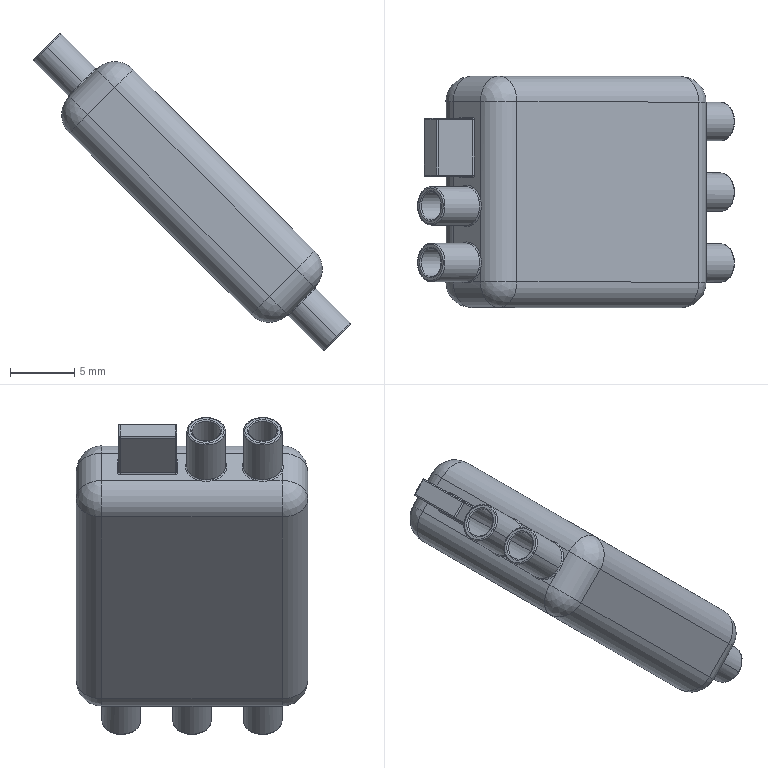Component | SolidWorks | 7.Electrical conector-1 | 1 solid | 148 faces | box 24.67 x 18 x 24.67 mm | volume 2959 mm3 | torus 50 | cylinder 44 | plane 29 | spline 13 | sphere 12 | commonest cylinder face diameters 4 x12 0.2 x12 2.2 x10 3 x10